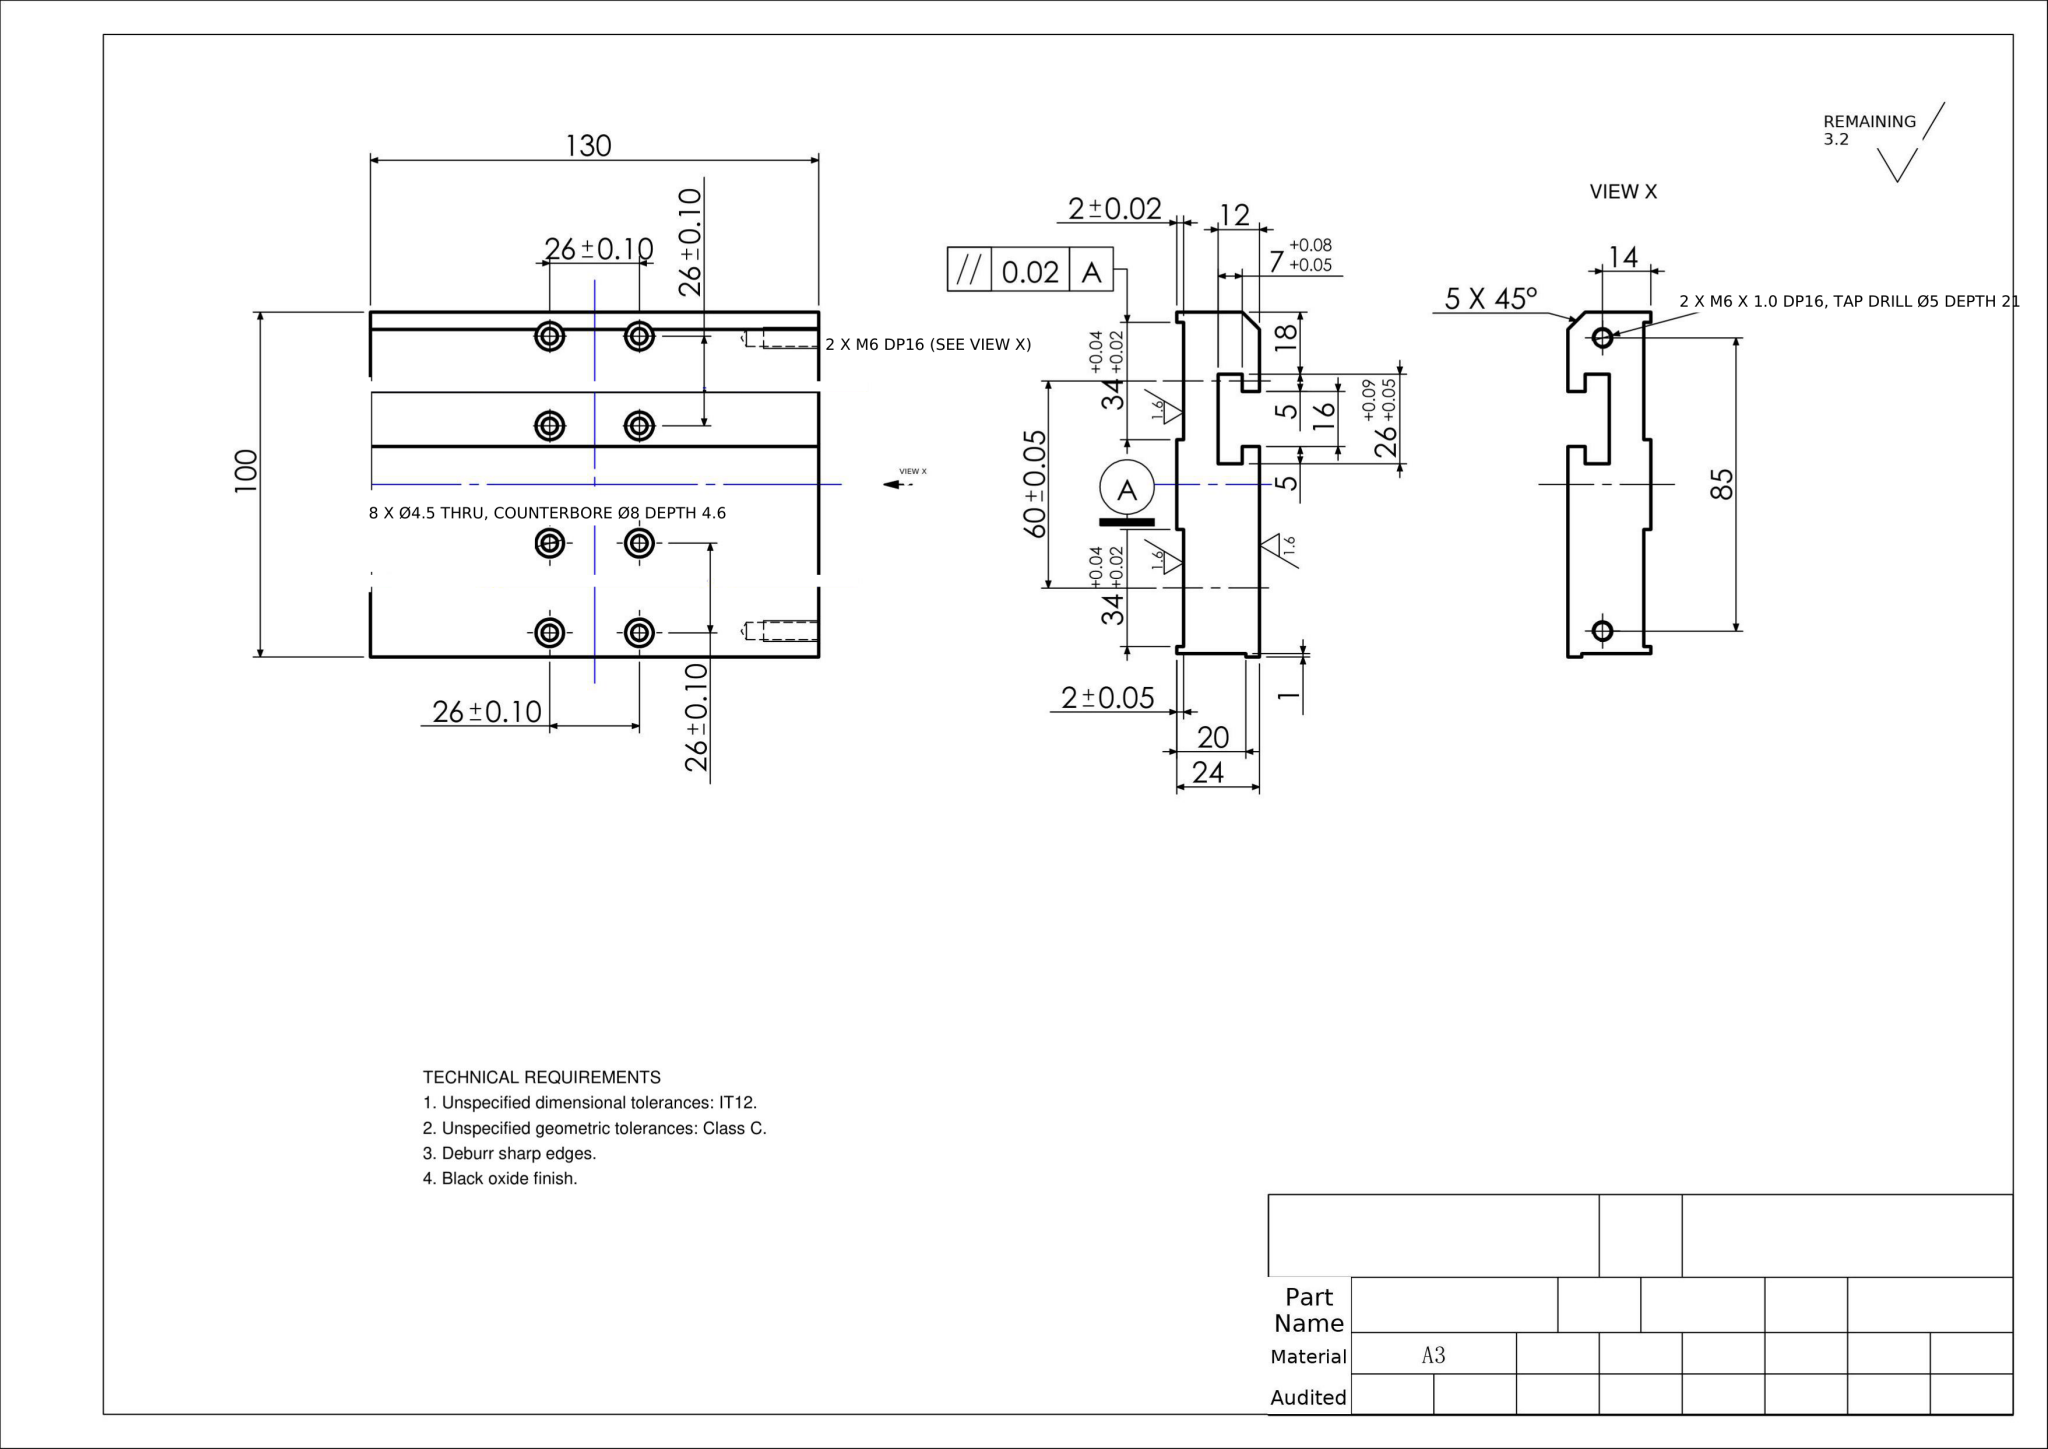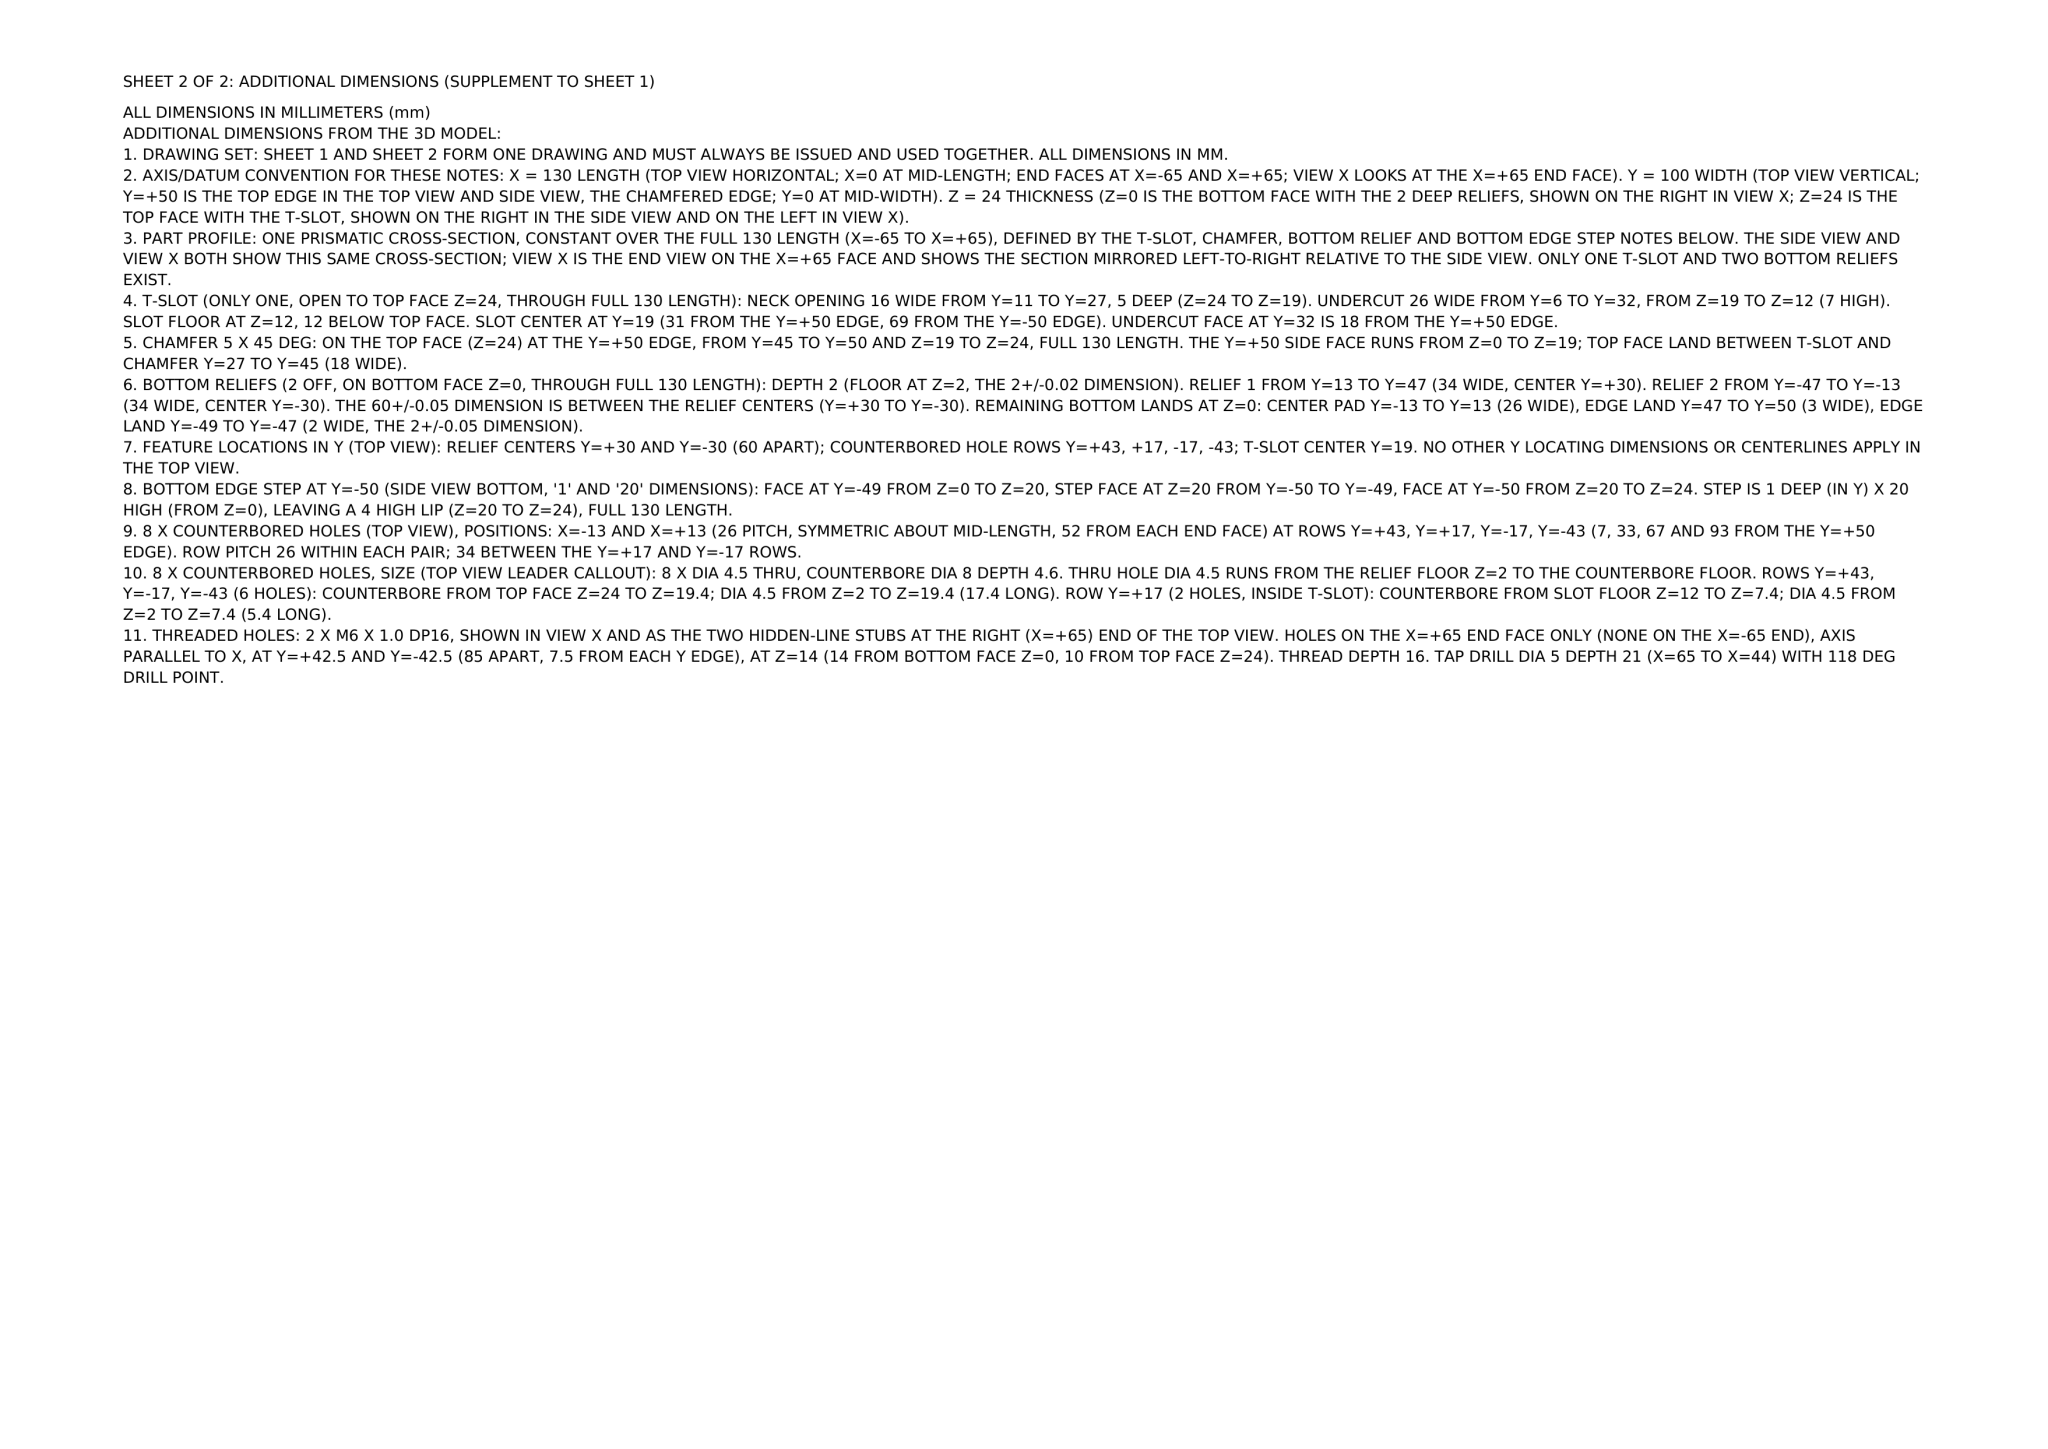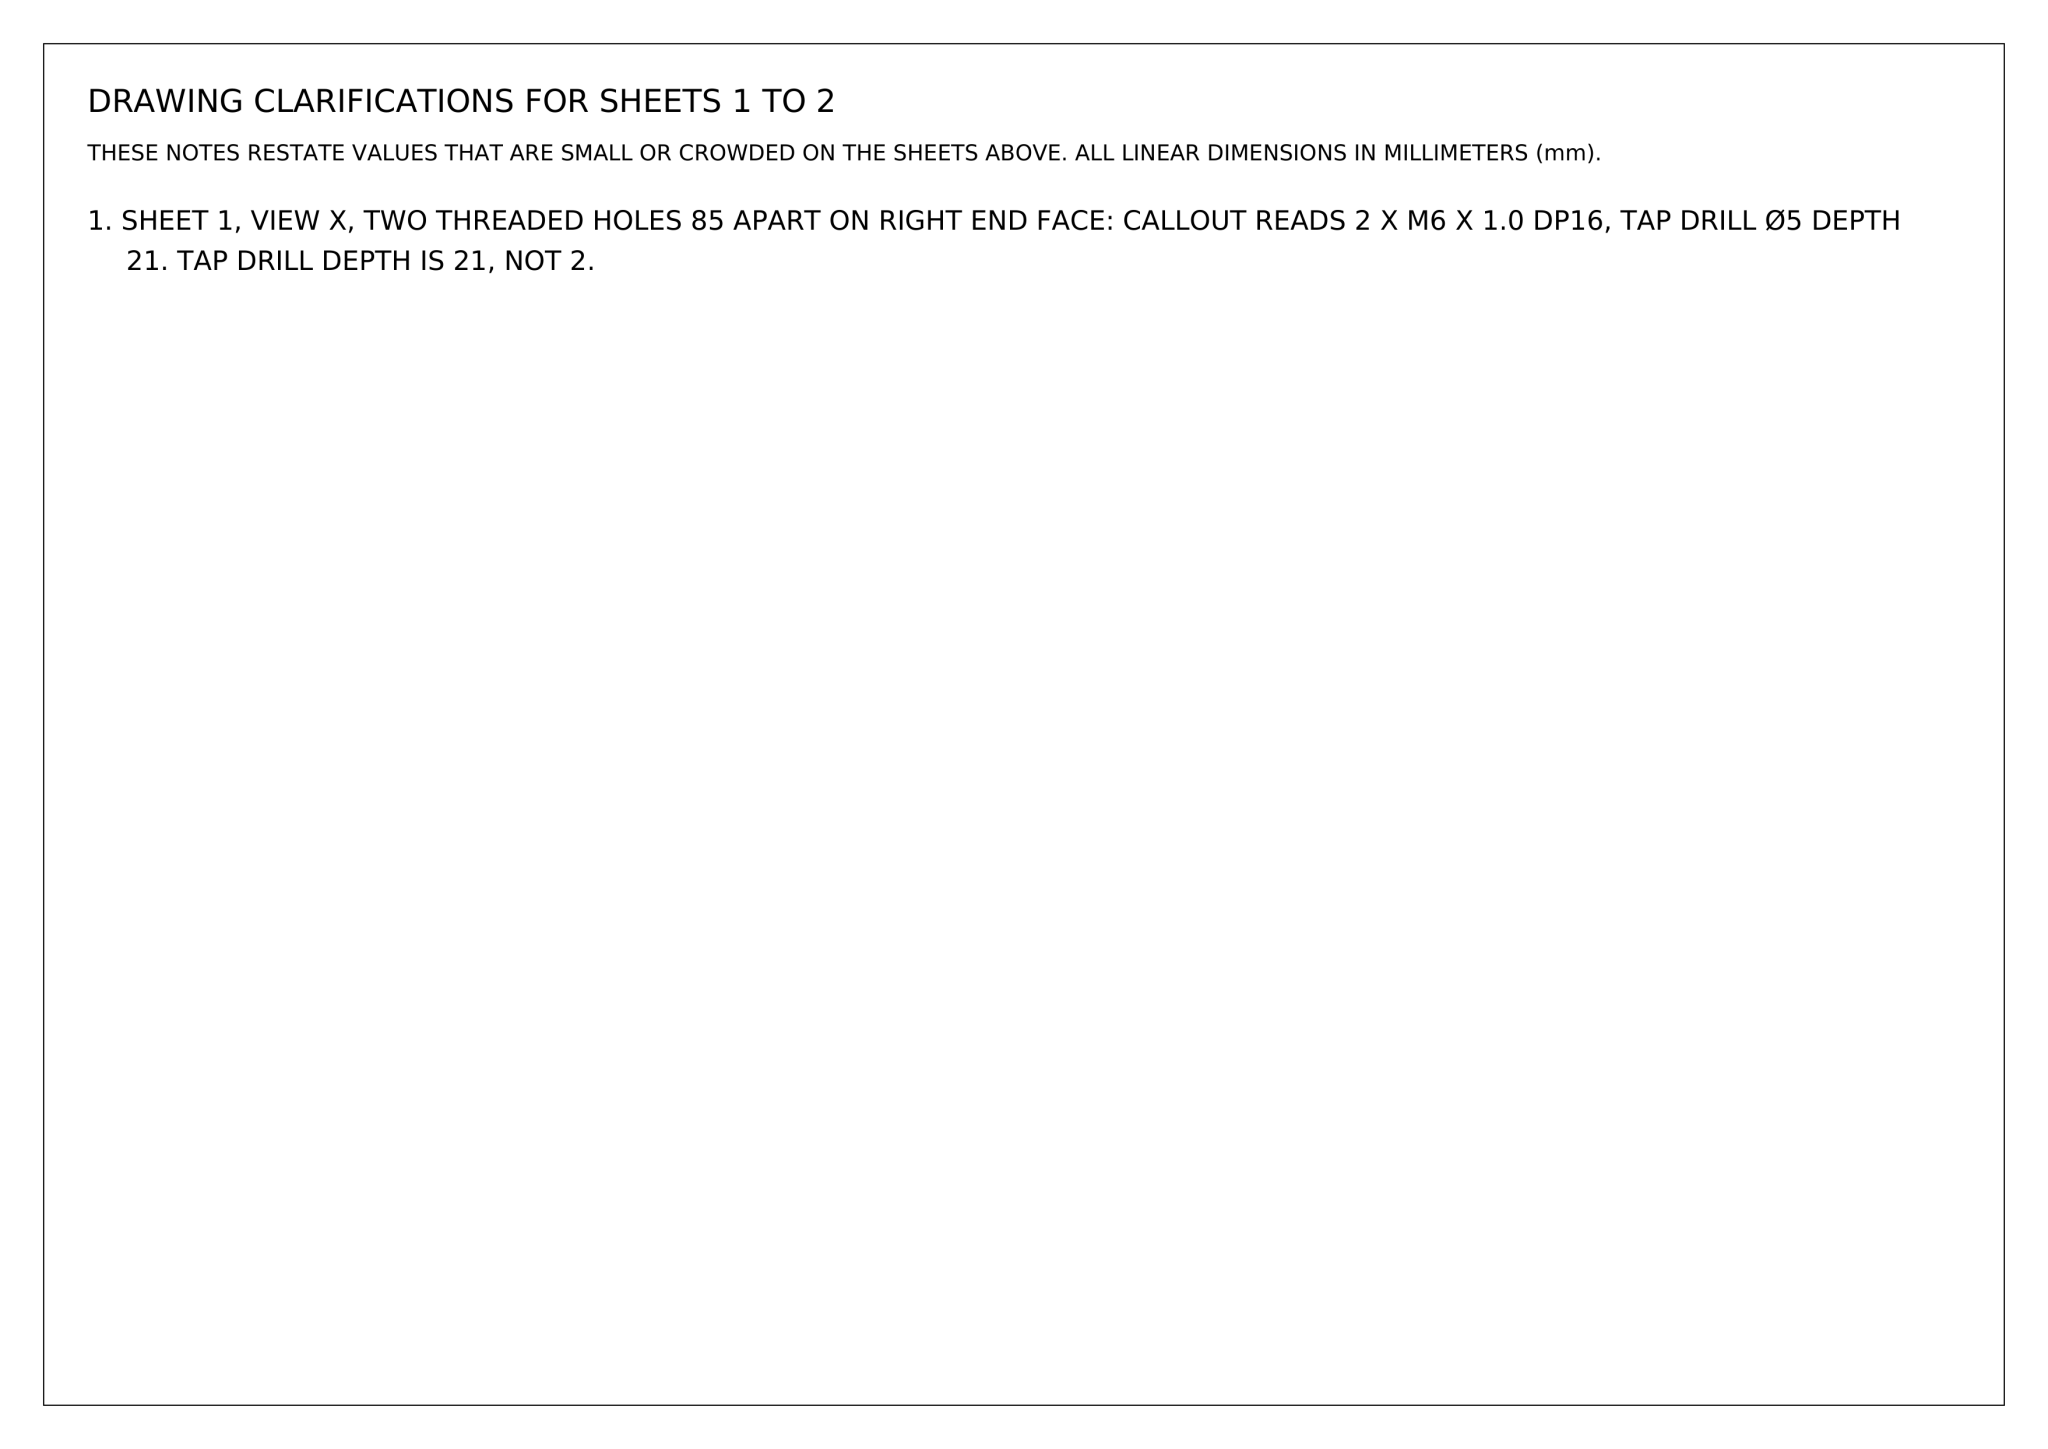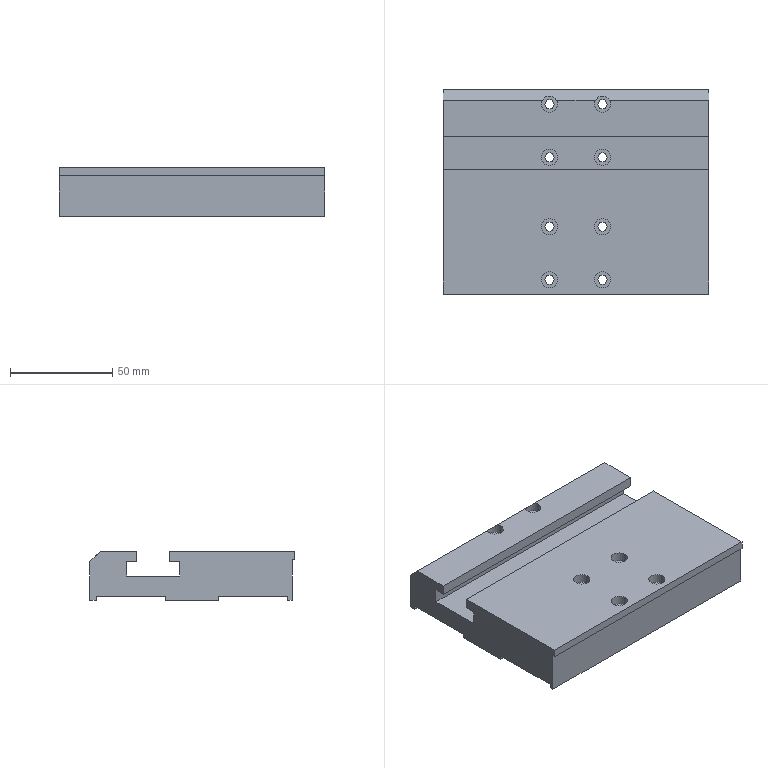Part | NX | mm | 1 solid | 73 faces | box 130 x 100 x 24 mm | volume 251525 mm3 | cylinder 36 | plane 33 | cone 4 | commonest cylinder face diameters 8 x16 4.5 x16 5 x4